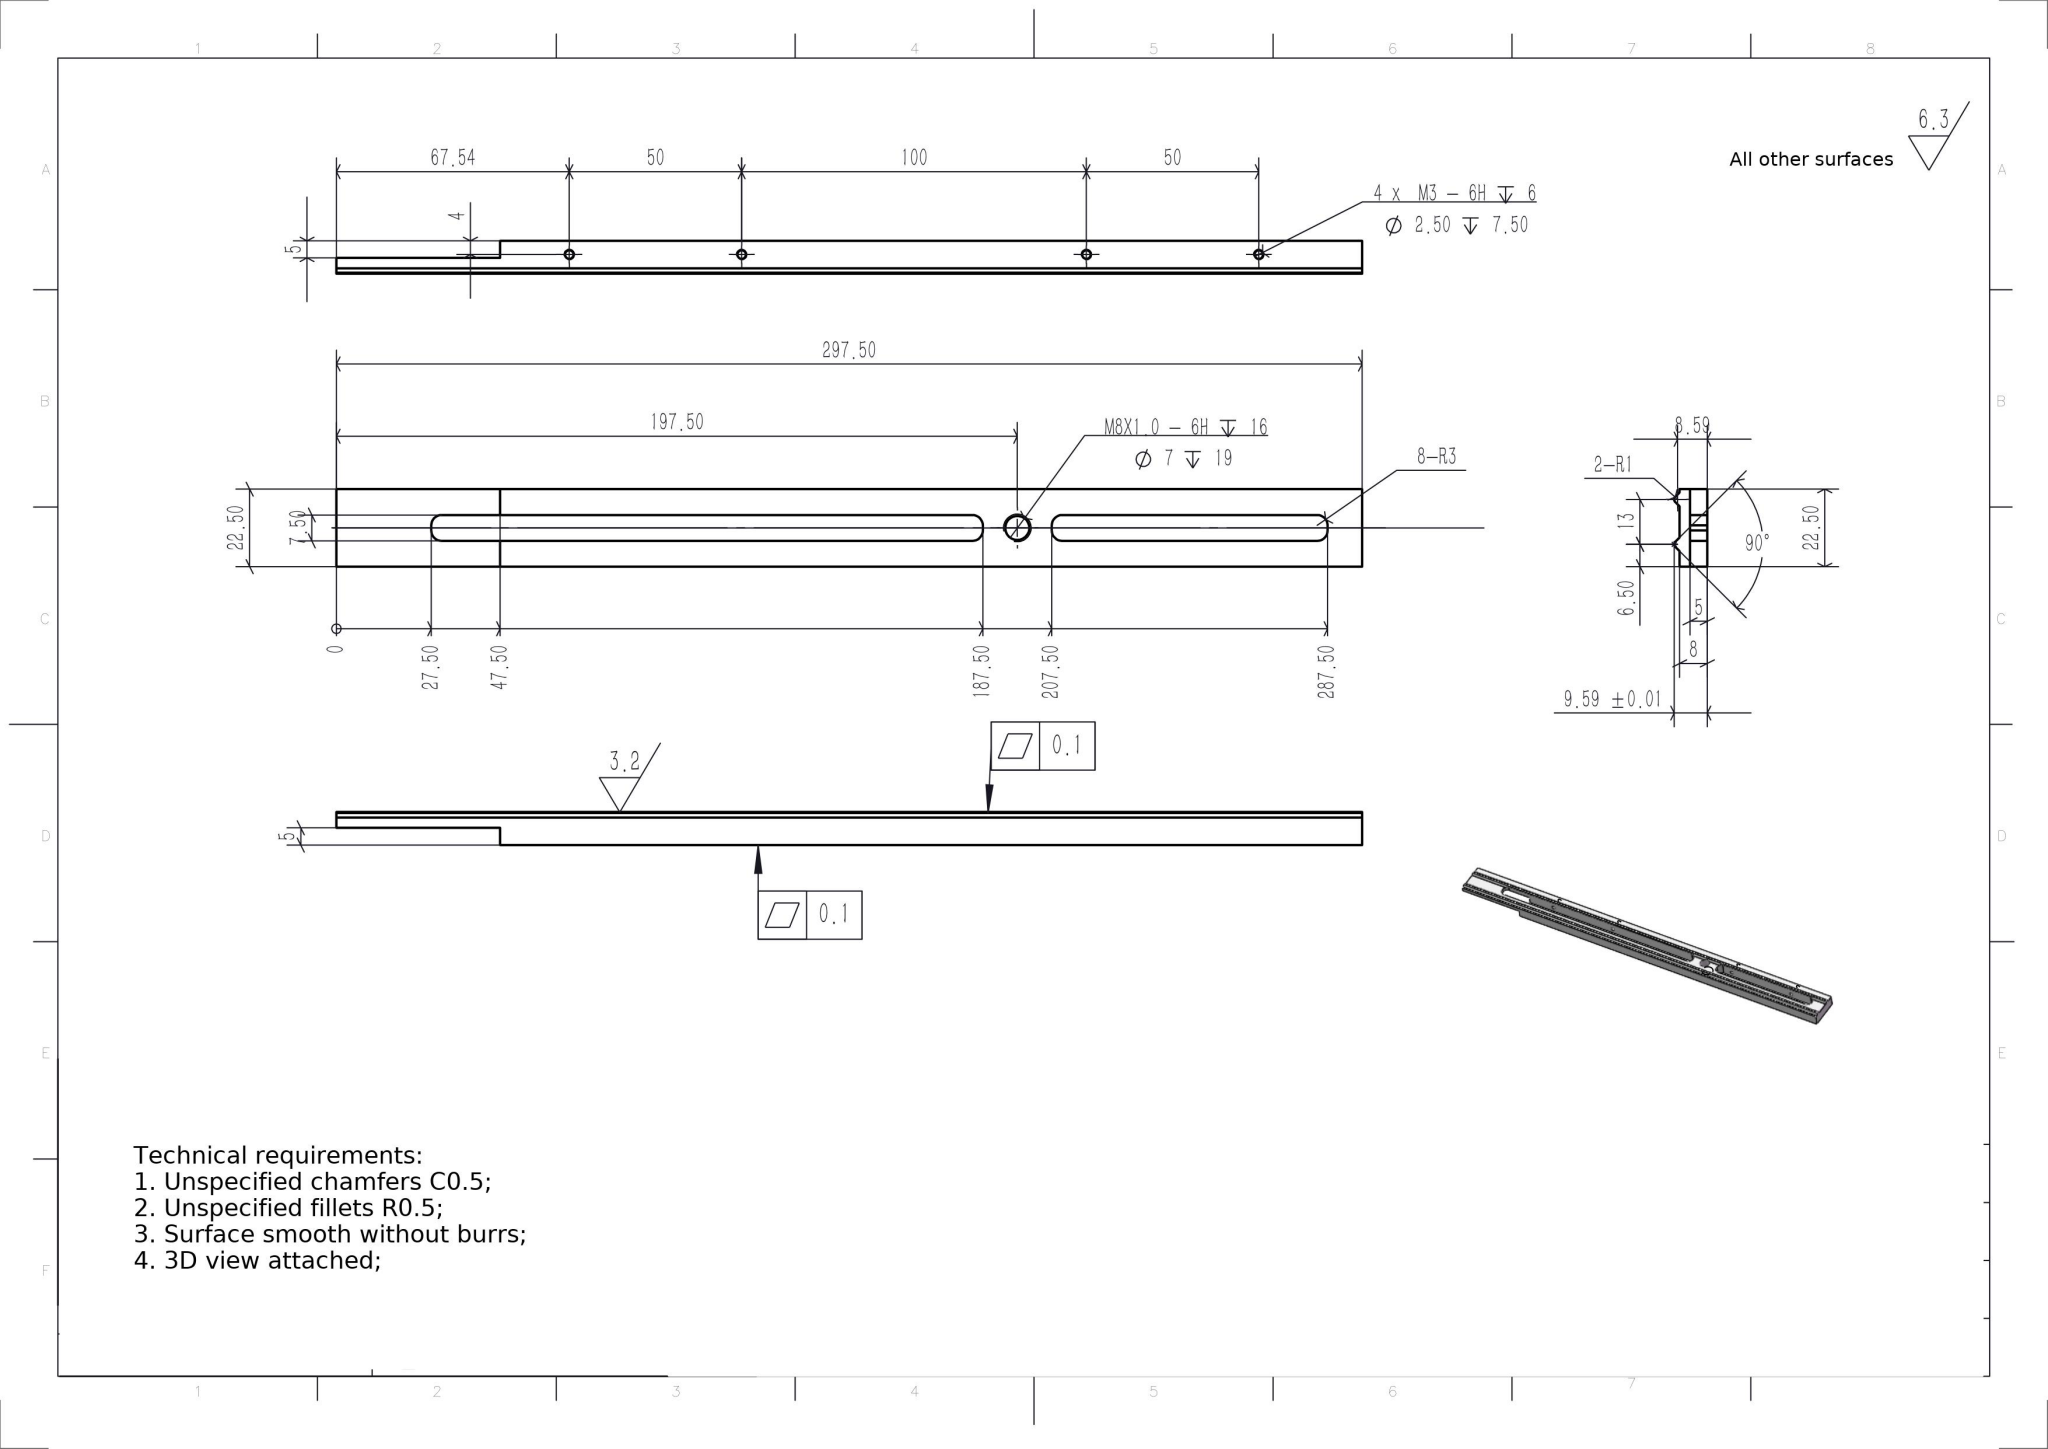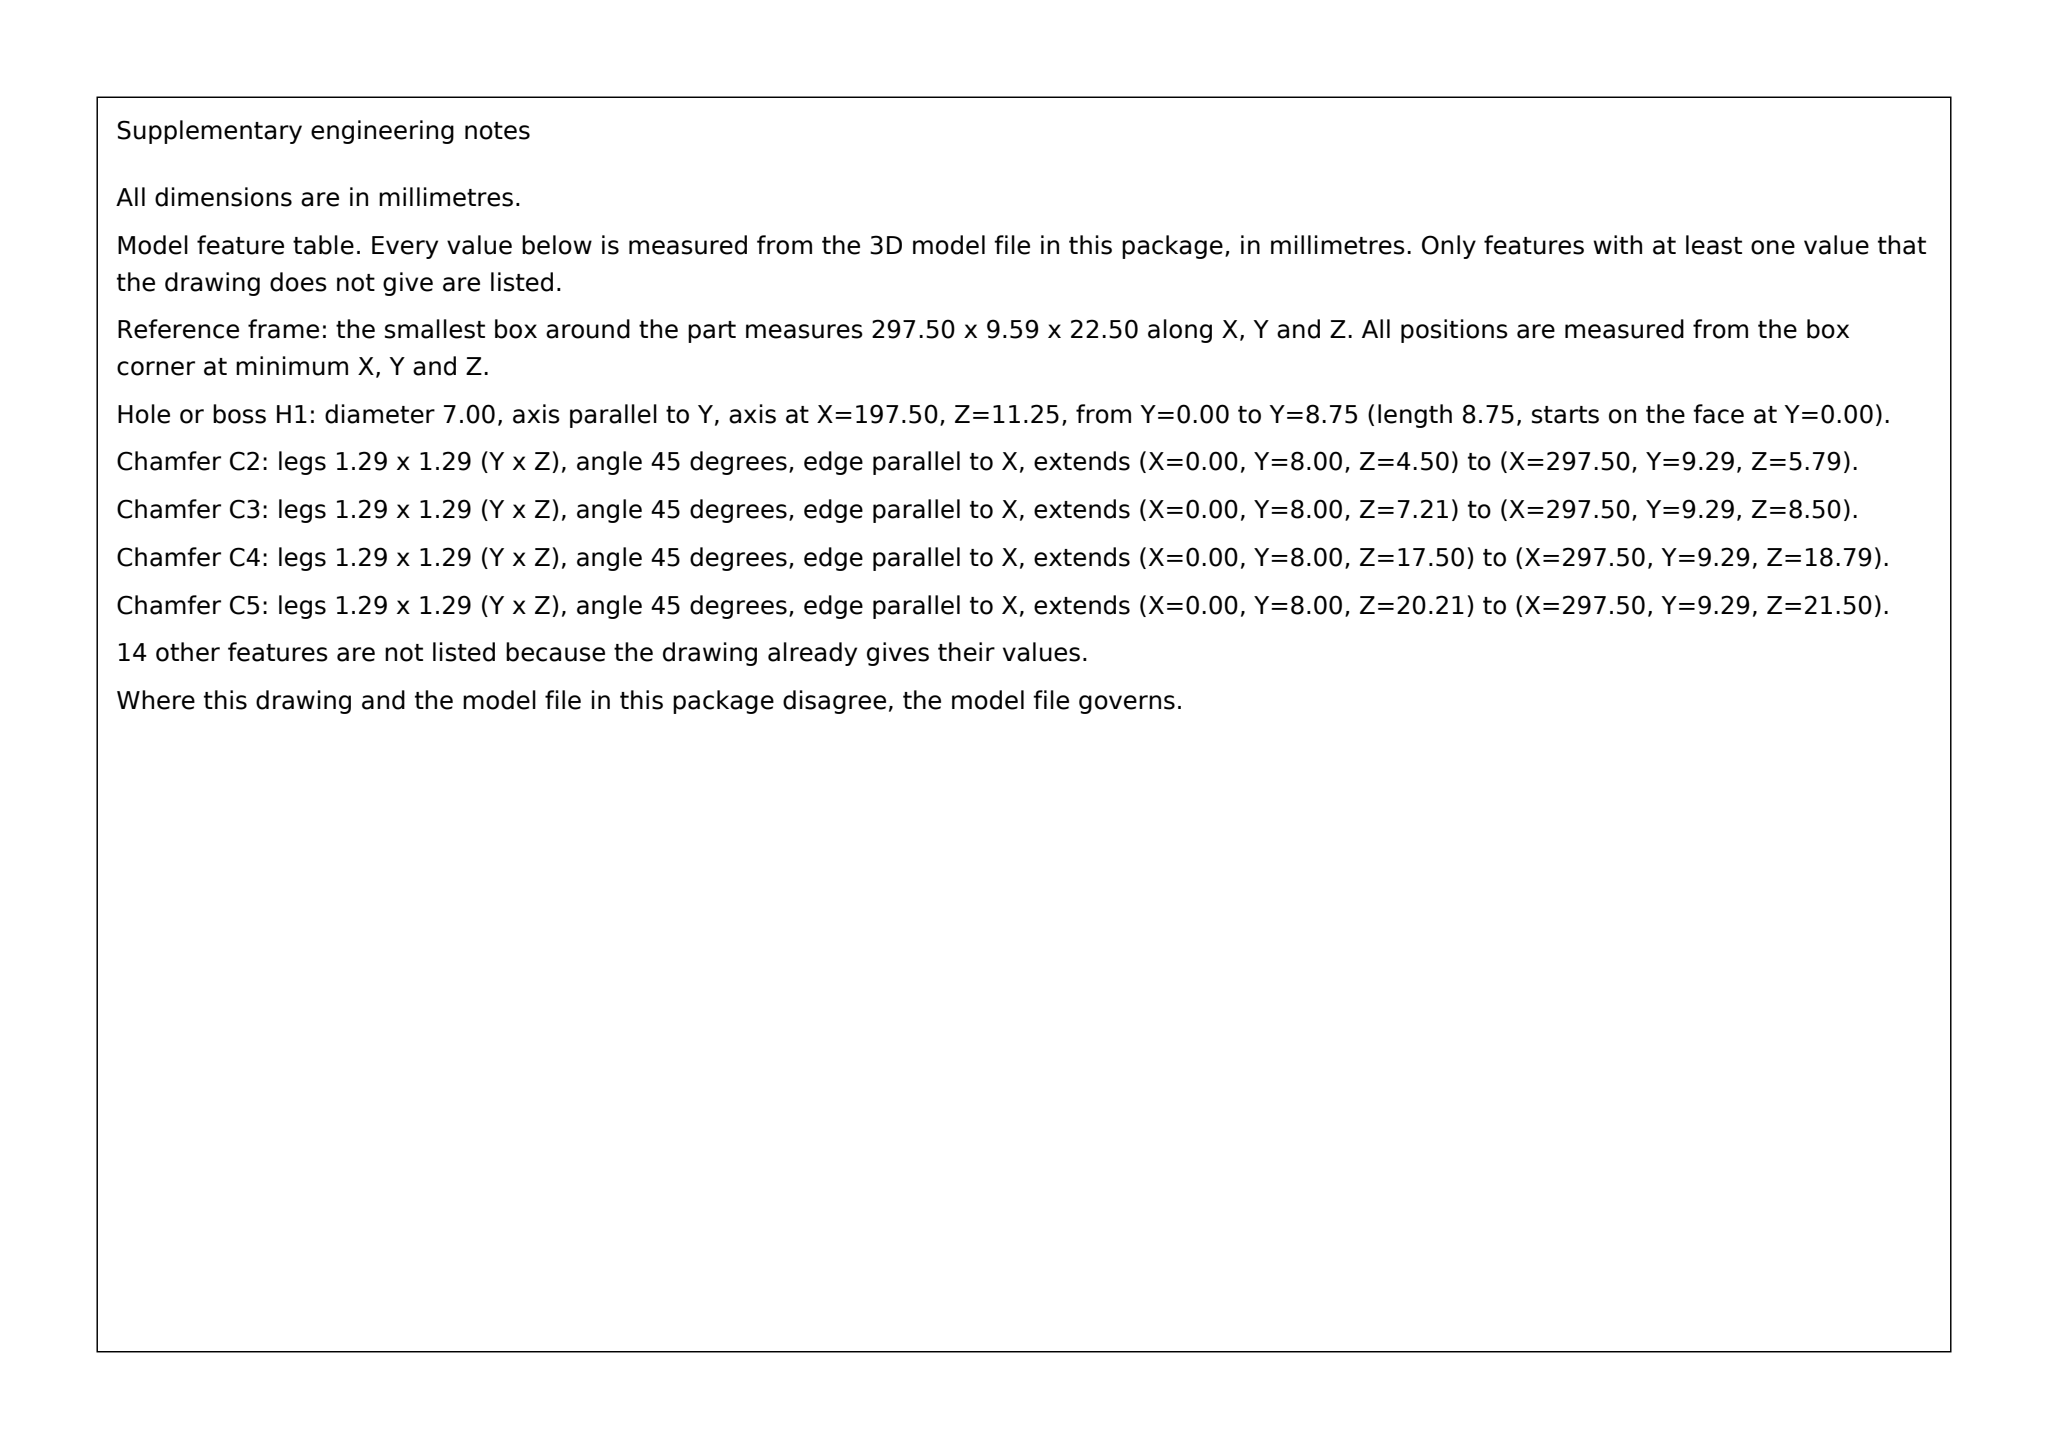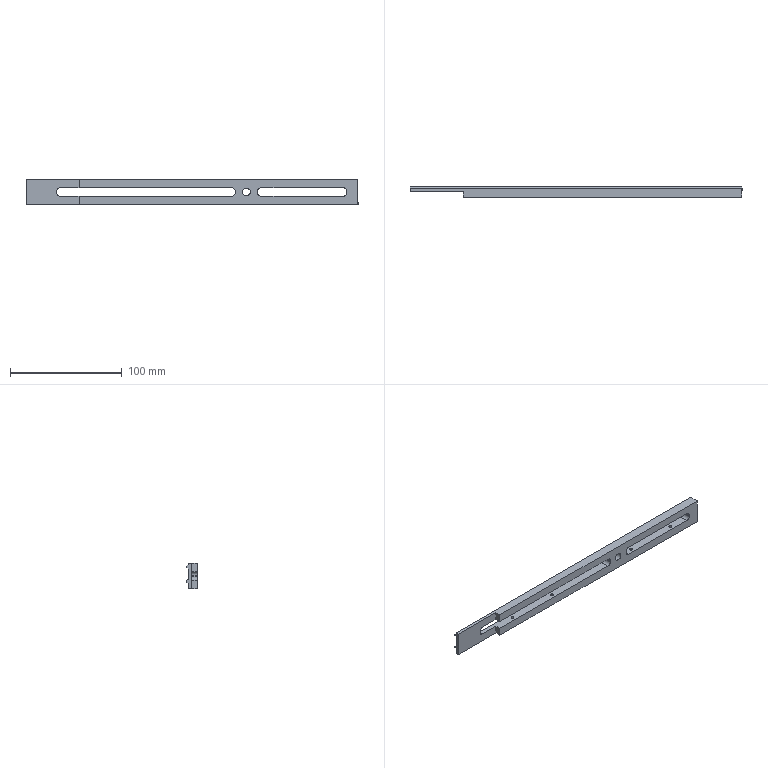Part | SolidWorks | mm | 1 solid | 43 faces | box 297.5 x 9.59 x 22.5 mm | volume 36341 mm3 | plane 23 | cylinder 20 | commonest cylinder face diameters 2.5 x8 6 x8 7 x2 2 x2
build123d program:
from build123d import *

# Parameters (mm, degrees)
SKETCH1_W                 = 300
SKETCH1_H                 = 22.5
BOSS_EXTRUDE1_DEPTH       = 10
CUT_EXTRUDE1_DEPTH        = 301.377
SKETCH4_W                 = 22.5
SKETCH4_H                 = 5
CUT_EXTRUDE3_DEPTH        = 50
M3_TAPPED_HOLE1_D         = 2.5
M3_TAPPED_HOLE1_DEPTH     = 7.5
M3_TAPPED_HOLE1_TIP       = 0.7511
M8X1_0_TAPPED_HOLE1_D     = 7
M8X1_0_TAPPED_HOLE1_DEPTH = 19
M8X1_0_TAPPED_HOLE1_TIP   = 2.103
CUT_EXTRUDE4_DEPTH        = 50
FILLET1_R                 = 1
SKETCH11_W                = 2.5
SKETCH11_H                = 22.5
CUT_EXTRUDE5_DEPTH        = 10


with BuildPart() as part:
    # Sketch1 → Boss-Extrude1 (new body)
    with BuildSketch(Plane(origin=(0, 0, 0), x_dir=(1, 0, 0), z_dir=(0, 1, 0))):
        Rectangle(SKETCH1_W, SKETCH1_H)
    extrude(amount=BOSS_EXTRUDE1_DEPTH)

    # Sketch2 → Cut-Extrude1 (cut, through all)
    with BuildSketch(Plane.ZY.offset(150)):
        Polygon((-6.75, 8), (-4.75, 10), (-11.25, 10), (-11.25, 8), align=None)
        Polygon((6.25, 8), (8.25, 10), (-4.75, 10), (-2.75, 8), align=None)
        Polygon((11.25, 10), (8.25, 10), (10.25, 8), (11.25, 8), align=None)
    extrude(amount=-CUT_EXTRUDE1_DEPTH, mode=Mode.SUBTRACT)

    # Sketch4 → Cut-Extrude3 (cut)
    with BuildSketch(Plane.ZY.offset(150)):
        with Locations((0, 2.5)):
            Rectangle(SKETCH4_W, SKETCH4_H)
    extrude(amount=-CUT_EXTRUDE3_DEPTH, mode=Mode.SUBTRACT)

    # M3 Tapped Hole1
    with Locations(Plane(origin=(0, 0, -11.25), x_dir=(-1, 0, 0), z_dir=(0, 0, -1))):
        with Locations((-120.04, 3.996), (-70.04, 3.996), (29.96, 3.996), (79.96, 3.996)):
            Hole(M3_TAPPED_HOLE1_D / 2, depth=M3_TAPPED_HOLE1_DEPTH)
            with Locations((0, 0, -(M3_TAPPED_HOLE1_DEPTH + M3_TAPPED_HOLE1_TIP / 2))):  # 118° drill point
                Cone(0, M3_TAPPED_HOLE1_D / 2, M3_TAPPED_HOLE1_TIP, mode=Mode.SUBTRACT)

    # M8x1.0 Tapped Hole1
    with Locations(Plane(origin=(0, 0, 0), x_dir=(-1, 0, 0), z_dir=(0, -1, 0))):
        with Locations((-50, 0)):
            Hole(M8X1_0_TAPPED_HOLE1_D / 2, depth=M8X1_0_TAPPED_HOLE1_DEPTH)
            with Locations((0, 0, -(M8X1_0_TAPPED_HOLE1_DEPTH + M8X1_0_TAPPED_HOLE1_TIP / 2))):  # 118° drill point
                Cone(0, M8X1_0_TAPPED_HOLE1_D / 2, M8X1_0_TAPPED_HOLE1_TIP, mode=Mode.SUBTRACT)

    # Sketch9 → Cut-Extrude4 (cut)
    with BuildSketch(Plane.XZ):
        with BuildLine():
            Line((63, 3.75), (137, 3.75))
            ThreePointArc((137, 3.75), (139.121, 2.871), (140, 0.75))
            Line((140, 0.75), (140, -0.75))
            ThreePointArc((140, -0.75), (139.121, -2.871), (137, -3.75))
            Line((137, -3.75), (63, -3.75))
            ThreePointArc((63, -3.75), (60.879, -2.871), (60, -0.75))
            Line((60, -0.75), (60, 0.75))
            ThreePointArc((60, 0.75), (60.879, 2.871), (63, 3.75))
        make_face()
        with BuildLine():
            Line((-117, 3.75), (37, 3.75))
            ThreePointArc((37, 3.75), (39.121, 2.871), (40, 0.75))
            Line((40, 0.75), (40, -0.75))
            ThreePointArc((40, -0.75), (39.121, -2.871), (37, -3.75))
            Line((37, -3.75), (-117, -3.75))
            ThreePointArc((-117, -3.75), (-119.121, -2.871), (-120, -0.75))
            Line((-120, -0.75), (-120, 0.75))
            ThreePointArc((-120, 0.75), (-119.121, 2.871), (-117, 3.75))
        make_face()
    extrude(amount=-CUT_EXTRUDE4_DEPTH, mode=Mode.SUBTRACT)

    # Fillet1
    fillet1_edges = [part.edges().sort_by_distance(p)[0] for p in [
        (0, 10, -4.75),
        (0, 10, 8.25),
    ]]
    fillet(fillet1_edges, radius=FILLET1_R)

    # Sketch11 → Cut-Extrude5 (cut)
    with BuildSketch(Plane.XZ.offset(-5)):
        with Locations((-148.75, 0)):
            Rectangle(SKETCH11_W, SKETCH11_H)
    extrude(amount=-CUT_EXTRUDE5_DEPTH, mode=Mode.SUBTRACT)


solid = part.part